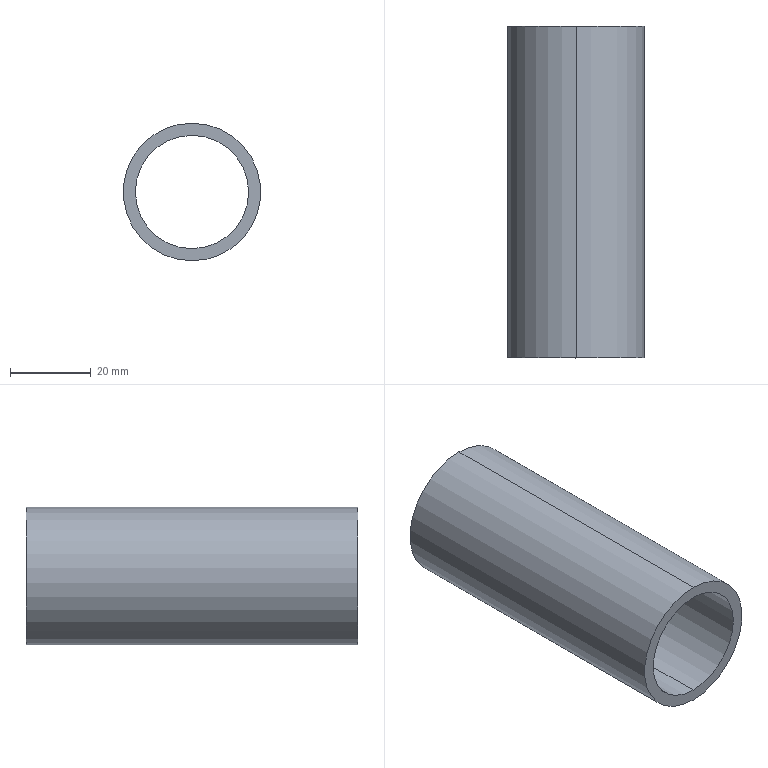Component | SolidWorks | CCQ-1.1-9WeldedPipe-1 | 1 solid | 6 faces | box 34 x 82 x 34 mm | volume 23958 mm3 | cylinder 4 | plane 2 | commonest cylinder face diameters 34 x2 28 x2 | material 304
build123d program:
from build123d import *

# Parameters (mm, degrees)
SKETCH1_R                      = 17
SKETCH1_R_2                    = 14
WELDED_STEEL_PIPE_34X3_1_DEPTH = 82


with BuildPart() as part:
    # Sketch1 → Welded Steel Pipe _34X3_1 (new body)
    with BuildSketch(Plane.YZ.offset(-41)):
        Circle(SKETCH1_R)
        Circle(SKETCH1_R_2, mode=Mode.SUBTRACT)
    extrude(amount=WELDED_STEEL_PIPE_34X3_1_DEPTH)


solid = part.part

# Placed as in the assembly
solid = solid.moved(Location((20, -499.5, 0), (0, 0, 90)))
STEP:
#1=COLOUR_RGB('',0.7922,0.8196,0.9333);
#2=FILL_AREA_STYLE_COLOUR('',#1);
#3=FILL_AREA_STYLE('',(#2));
#4=SURFACE_STYLE_FILL_AREA(#3);
#5=SURFACE_SIDE_STYLE('',(#4));
#6=SURFACE_STYLE_USAGE(.BOTH.,#5);
#7=PRESENTATION_STYLE_ASSIGNMENT((#6));
#8=CARTESIAN_POINT('',(0.7913,-21.28,0.6693));
#9=VERTEX_POINT('',#8);
#10=CARTESIAN_POINT('',(0.7835,-21.28,-0.6693));
#11=VERTEX_POINT('',#10);
#12=CARTESIAN_POINT('',(0.7874,-21.28,-0.));
#13=DIRECTION('',(0.,-1.,-0.));
#14=DIRECTION('',(0.005805,0.,1.));
#15=AXIS2_PLACEMENT_3D('',#12,#13,#14);
#16=CIRCLE('',#15,0.6693);
#17=EDGE_CURVE('',#9,#11,#16,.T.);
#18=ORIENTED_EDGE('',*,*,#17,.F.);
#19=CARTESIAN_POINT('',(0.7913,-18.051,0.6693));
#20=VERTEX_POINT('',#19);
#21=CARTESIAN_POINT('',(0.7913,-21.28,0.6693));
#22=DIRECTION('',(-0.,1.,0.));
#23=VECTOR('',#22,39.37);
#24=LINE('',#21,#23);
#25=EDGE_CURVE('',#9,#20,#24,.T.);
#26=ORIENTED_EDGE('',*,*,#25,.T.);
#27=CARTESIAN_POINT('',(0.7835,-18.051,-0.6693));
#28=VERTEX_POINT('',#27);
#29=CARTESIAN_POINT('',(0.7874,-18.051,-0.));
#30=DIRECTION('',(0.,-1.,-0.));
#31=DIRECTION('',(0.005805,0.,1.));
#32=AXIS2_PLACEMENT_3D('',#29,#30,#31);
#33=CIRCLE('',#32,0.6693);
#34=EDGE_CURVE('',#20,#28,#33,.T.);
#35=ORIENTED_EDGE('',*,*,#34,.T.);
#36=CARTESIAN_POINT('',(0.7835,-21.28,-0.6693));
#37=DIRECTION('',(-0.,1.,0.));
#38=VECTOR('',#37,39.37);
#39=LINE('',#36,#38);
#40=EDGE_CURVE('',#11,#28,#39,.T.);
#41=ORIENTED_EDGE('',*,*,#40,.F.);
#42=EDGE_LOOP('',(#18,#26,#35,#41));
#43=FACE_OUTER_BOUND('',#42,.T.);
#44=CARTESIAN_POINT('',(0.7874,-21.28,-0.));
#45=DIRECTION('',(-0.,1.,0.));
#46=DIRECTION('',(-0.005805,0.,-1.));
#47=AXIS2_PLACEMENT_3D('',#44,#45,#46);
#48=CYLINDRICAL_SURFACE('',#47,0.6693);
#49=ADVANCED_FACE('',(#43),#48,.T.);
#50=CARTESIAN_POINT('',(0.7842,-21.28,-0.5512));
#51=VERTEX_POINT('',#50);
#52=CARTESIAN_POINT('',(0.7906,-21.28,0.5512));
#53=VERTEX_POINT('',#52);
#54=CARTESIAN_POINT('',(0.7874,-21.28,-0.));
#55=DIRECTION('',(0.,-1.,-0.));
#56=DIRECTION('',(0.005805,0.,1.));
#57=AXIS2_PLACEMENT_3D('',#54,#55,#56);
#58=CIRCLE('',#57,0.5512);
#59=EDGE_CURVE('',#51,#53,#58,.T.);
#60=ORIENTED_EDGE('',*,*,#59,.T.);
#61=CARTESIAN_POINT('',(0.7906,-18.051,0.5512));
#62=VERTEX_POINT('',#61);
#63=CARTESIAN_POINT('',(0.7906,-21.28,0.5512));
#64=DIRECTION('',(-0.,1.,0.));
#65=VECTOR('',#64,39.37);
#66=LINE('',#63,#65);
#67=EDGE_CURVE('',#53,#62,#66,.T.);
#68=ORIENTED_EDGE('',*,*,#67,.T.);
#69=CARTESIAN_POINT('',(0.7842,-18.051,-0.5512));
#70=VERTEX_POINT('',#69);
#71=CARTESIAN_POINT('',(0.7874,-18.051,-0.));
#72=DIRECTION('',(0.,-1.,-0.));
#73=DIRECTION('',(0.005805,0.,1.));
#74=AXIS2_PLACEMENT_3D('',#71,#72,#73);
#75=CIRCLE('',#74,0.5512);
#76=EDGE_CURVE('',#70,#62,#75,.T.);
#77=ORIENTED_EDGE('',*,*,#76,.F.);
#78=CARTESIAN_POINT('',(0.7842,-21.28,-0.5512));
#79=DIRECTION('',(-0.,1.,0.));
#80=VECTOR('',#79,39.37);
#81=LINE('',#78,#80);
#82=EDGE_CURVE('',#51,#70,#81,.T.);
#83=ORIENTED_EDGE('',*,*,#82,.F.);
#84=EDGE_LOOP('',(#60,#68,#77,#83));
#85=FACE_OUTER_BOUND('',#84,.T.);
#86=CARTESIAN_POINT('',(0.7874,-21.28,-0.));
#87=DIRECTION('',(-0.,1.,0.));
#88=DIRECTION('',(-0.005805,0.,-1.));
#89=AXIS2_PLACEMENT_3D('',#86,#87,#88);
#90=CYLINDRICAL_SURFACE('',#89,0.5512);
#91=ADVANCED_FACE('',(#85),#90,.F.);
#92=ORIENTED_EDGE('',*,*,#67,.F.);
#93=CARTESIAN_POINT('',(0.7874,-21.28,-0.));
#94=DIRECTION('',(0.,-1.,-0.));
#95=DIRECTION('',(0.005805,0.,1.));
#96=AXIS2_PLACEMENT_3D('',#93,#94,#95);
#97=CIRCLE('',#96,0.5512);
#98=EDGE_CURVE('',#53,#51,#97,.T.);
#99=ORIENTED_EDGE('',*,*,#98,.T.);
#100=ORIENTED_EDGE('',*,*,#82,.T.);
#101=CARTESIAN_POINT('',(0.7874,-18.051,-0.));
#102=DIRECTION('',(0.,-1.,-0.));
#103=DIRECTION('',(0.005805,0.,1.));
#104=AXIS2_PLACEMENT_3D('',#101,#102,#103);
#105=CIRCLE('',#104,0.5512);
#106=EDGE_CURVE('',#62,#70,#105,.T.);
#107=ORIENTED_EDGE('',*,*,#106,.F.);
#108=EDGE_LOOP('',(#92,#99,#100,#107));
#109=FACE_OUTER_BOUND('',#108,.T.);
#110=CARTESIAN_POINT('',(0.7874,-21.28,-0.));
#111=DIRECTION('',(-0.,1.,0.));
#112=DIRECTION('',(-0.005805,0.,-1.));
#113=AXIS2_PLACEMENT_3D('',#110,#111,#112);
#114=CYLINDRICAL_SURFACE('',#113,0.5512);
#115=ADVANCED_FACE('',(#109),#114,.F.);
#116=ORIENTED_EDGE('',*,*,#25,.F.);
#117=CARTESIAN_POINT('',(0.7874,-21.28,-0.));
#118=DIRECTION('',(0.,-1.,-0.));
#119=DIRECTION('',(0.005805,0.,1.));
#120=AXIS2_PLACEMENT_3D('',#117,#118,#119);
#121=CIRCLE('',#120,0.6693);
#122=EDGE_CURVE('',#11,#9,#121,.T.);
#123=ORIENTED_EDGE('',*,*,#122,.F.);
#124=ORIENTED_EDGE('',*,*,#40,.T.);
#125=CARTESIAN_POINT('',(0.7874,-18.051,-0.));
#126=DIRECTION('',(0.,-1.,-0.));
#127=DIRECTION('',(0.005805,0.,1.));
#128=AXIS2_PLACEMENT_3D('',#125,#126,#127);
#129=CIRCLE('',#128,0.6693);
#130=EDGE_CURVE('',#28,#20,#129,.T.);
#131=ORIENTED_EDGE('',*,*,#130,.T.);
#132=EDGE_LOOP('',(#116,#123,#124,#131));
#133=FACE_OUTER_BOUND('',#132,.T.);
#134=CARTESIAN_POINT('',(0.7874,-21.28,-0.));
#135=DIRECTION('',(-0.,1.,0.));
#136=DIRECTION('',(-0.005805,0.,-1.));
#137=AXIS2_PLACEMENT_3D('',#134,#135,#136);
#138=CYLINDRICAL_SURFACE('',#137,0.6693);
#139=ADVANCED_FACE('',(#133),#138,.T.);
#140=ORIENTED_EDGE('',*,*,#59,.F.);
#141=ORIENTED_EDGE('',*,*,#98,.F.);
#142=EDGE_LOOP('',(#140,#141));
#143=FACE_BOUND('',#142,.T.);
#144=ORIENTED_EDGE('',*,*,#122,.T.);
#145=ORIENTED_EDGE('',*,*,#17,.T.);
#146=EDGE_LOOP('',(#144,#145));
#147=FACE_OUTER_BOUND('',#146,.T.);
#148=CARTESIAN_POINT('',(0.7874,-21.28,-0.));
#149=DIRECTION('',(0.,-1.,0.));
#150=DIRECTION('',(0.005805,0.,1.));
#151=AXIS2_PLACEMENT_3D('',#148,#149,#150);
#152=PLANE('',#151);
#153=ADVANCED_FACE('',(#143,#147),#152,.T.);
#154=ORIENTED_EDGE('',*,*,#76,.T.);
#155=ORIENTED_EDGE('',*,*,#106,.T.);
#156=EDGE_LOOP('',(#154,#155));
#157=FACE_BOUND('',#156,.T.);
#158=ORIENTED_EDGE('',*,*,#130,.F.);
#159=ORIENTED_EDGE('',*,*,#34,.F.);
#160=EDGE_LOOP('',(#158,#159));
#161=FACE_OUTER_BOUND('',#160,.T.);
#162=CARTESIAN_POINT('',(0.7874,-18.051,-0.));
#163=DIRECTION('',(0.,-1.,0.));
#164=DIRECTION('',(0.005805,0.,1.));
#165=AXIS2_PLACEMENT_3D('',#162,#163,#164);
#166=PLANE('',#165);
#167=ADVANCED_FACE('',(#157,#161),#166,.F.);
#168=CLOSED_SHELL('',(#49,#91,#115,#139,#153,#167));
#169=MANIFOLD_SOLID_BREP('',#168);
#170=STYLED_ITEM('',(#7),#169);
#171=(LENGTH_UNIT()NAMED_UNIT(*)SI_UNIT($,.METRE.));
#172=LENGTH_MEASURE_WITH_UNIT(LENGTH_MEASURE(0.0254),#171);
#173=DIMENSIONAL_EXPONENTS(1.,0.,0.,0.,0.,0.,0.);
#174=(CONVERSION_BASED_UNIT('',#172)LENGTH_UNIT()NAMED_UNIT(#173));
#175=UNCERTAINTY_MEASURE_WITH_UNIT(LENGTH_MEASURE(0.00001),#174,'','');
#176=(NAMED_UNIT(*)PLANE_ANGLE_UNIT()SI_UNIT($,.RADIAN.));
#177=(NAMED_UNIT(*)SI_UNIT($,.STERADIAN.)SOLID_ANGLE_UNIT());
#178=(GEOMETRIC_REPRESENTATION_CONTEXT(3)GLOBAL_UNCERTAINTY_ASSIGNED_CONTEXT((#175))GLOBAL_UNIT_ASSIGNED_CONTEXT((#174,#176,#177))REPRESENTATION_CONTEXT('',''));
#179=MECHANICAL_DESIGN_GEOMETRIC_PRESENTATION_REPRESENTATION('',(#170),#178);
#180=CARTESIAN_POINT('',(0.,0.,0.));
#181=DIRECTION('',(0.,0.,1.));
#182=DIRECTION('',(1.,0.,0.));
#183=AXIS2_PLACEMENT_3D('',#180,#181,#182);
#184=(LENGTH_UNIT()NAMED_UNIT(*)SI_UNIT($,.METRE.));
#185=LENGTH_MEASURE_WITH_UNIT(LENGTH_MEASURE(0.0254),#184);
#186=DIMENSIONAL_EXPONENTS(1.,0.,0.,0.,0.,0.,0.);
#187=(CONVERSION_BASED_UNIT('',#185)LENGTH_UNIT()NAMED_UNIT(#186));
#188=UNCERTAINTY_MEASURE_WITH_UNIT(LENGTH_MEASURE(0.00001),#187,'','');
#189=(NAMED_UNIT(*)PLANE_ANGLE_UNIT()SI_UNIT($,.RADIAN.));
#190=(NAMED_UNIT(*)SI_UNIT($,.STERADIAN.)SOLID_ANGLE_UNIT());
#191=(GEOMETRIC_REPRESENTATION_CONTEXT(3)GLOBAL_UNCERTAINTY_ASSIGNED_CONTEXT((#188))GLOBAL_UNIT_ASSIGNED_CONTEXT((#187,#189,#190))REPRESENTATION_CONTEXT('',''));
#192=ADVANCED_BREP_SHAPE_REPRESENTATION('',(#169,#183),#191);
#193=PRESENTATION_LAYER_ASSIGNMENT('','',(#170));